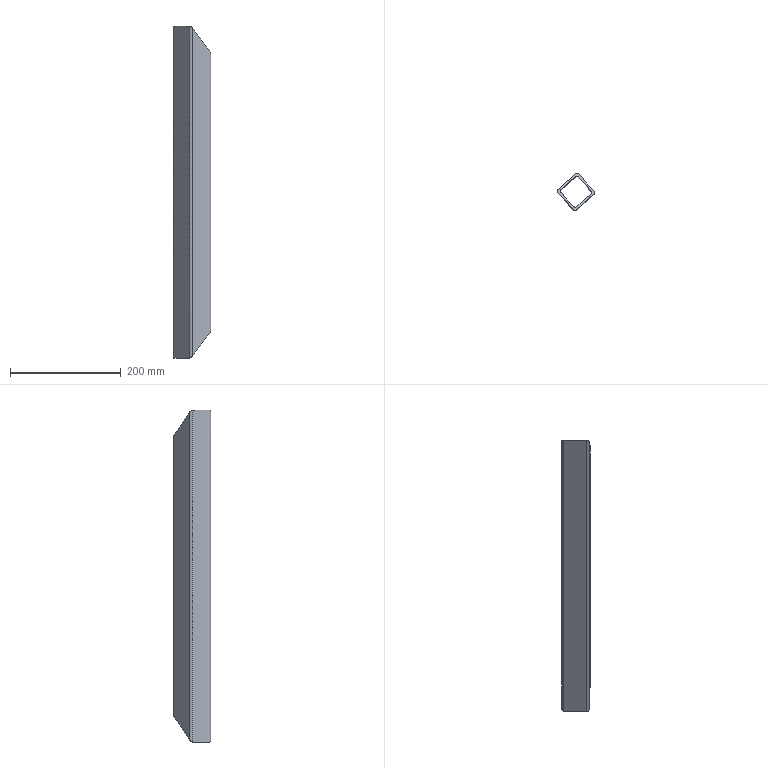Component | NX | ADJ_BRKT_BOT_BEAM | 1 solid | 18 faces | volume 404800 mm3 | plane 10 | cylinder 8 | commonest cylinder face diameters 8 x8